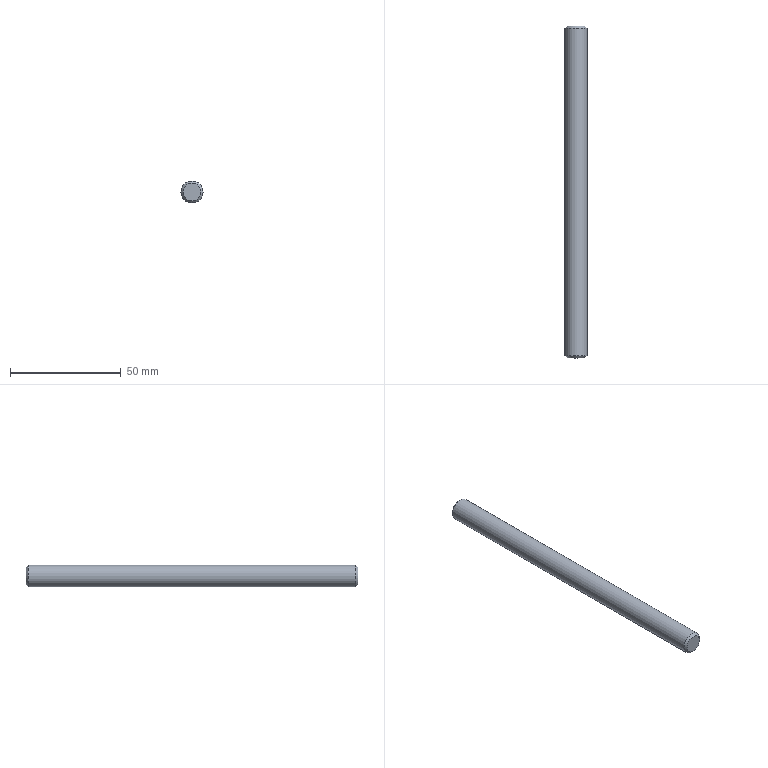Component | NX | REAMER_BAR | 1 solid | 5 faces | box 10 x 150 x 10 mm | volume 11752 mm3 | plane 2 | cone 2 | cylinder 1 | commonest cylinder face diameters 10 x1
STEP:
#1=CARTESIAN_POINT('',(0.,0.,0.));
#2=DIRECTION('',(0.,0.,1.));
#3=DIRECTION('',(1.,0.,0.));
#4=AXIS2_PLACEMENT_3D('',#1,#2,#3);
#5=CARTESIAN_POINT('',(-188.627,-125.996,15.));
#6=VERTEX_POINT('',#5);
#7=CARTESIAN_POINT('',(-192.627,-125.996,15.));
#8=DIRECTION('',(0.,-1.,0.));
#9=DIRECTION('',(1.,0.,0.));
#10=AXIS2_PLACEMENT_3D('',#7,#8,#9);
#11=CIRCLE('',#10,4.);
#12=CARTESIAN_POINT('',(-192.627,-125.996,15.));
#13=DIRECTION('',(0.,-1.,0.));
#14=DIRECTION('',(1.,0.,0.));
#15=AXIS2_PLACEMENT_3D('',#12,#13,#14);
#16=PLANE('',#15);
#17=CARTESIAN_POINT('',(0.,0.));
#18=DIRECTION('',(1.,0.));
#19=AXIS2_PLACEMENT_2D('',#17,#18);
#20=CIRCLE('',#19,4.);
#21=(GEOMETRIC_REPRESENTATION_CONTEXT(2)PARAMETRIC_REPRESENTATION_CONTEXT()REPRESENTATION_CONTEXT('',''));
#22=DEFINITIONAL_REPRESENTATION('',(#20),#21);
#23=PCURVE('',#16,#22);
#24=CARTESIAN_POINT('',(-192.627,-124.996,15.));
#25=DIRECTION('',(0.,1.,0.));
#26=DIRECTION('',(-1.,0.,0.));
#27=AXIS2_PLACEMENT_3D('',#24,#25,#26);
#28=CONICAL_SURFACE('',#27,5.,0.7854);
#29=CARTESIAN_POINT('',(9.425,-1.));
#30=DIRECTION('',(-1.,0.));
#31=VECTOR('',#30,1.);
#32=LINE('',#29,#31);
#33=(GEOMETRIC_REPRESENTATION_CONTEXT(2)PARAMETRIC_REPRESENTATION_CONTEXT()REPRESENTATION_CONTEXT('',''));
#34=DEFINITIONAL_REPRESENTATION('',(#32),#33);
#35=PCURVE('',#28,#34);
#36=SURFACE_CURVE('',#11,(#23,#35),.PCURVE_S1.);
#37=EDGE_CURVE('',#6,#6,#36,.T.);
#38=ORIENTED_EDGE('',*,*,#37,.T.);
#39=EDGE_LOOP('',(#38));
#40=FACE_BOUND('',#39,.T.);
#41=ADVANCED_FACE('',(#40),#16,.T.);
#42=CARTESIAN_POINT('',(-196.627,24.004,15.));
#43=VERTEX_POINT('',#42);
#44=CARTESIAN_POINT('',(-192.627,24.004,15.));
#45=DIRECTION('',(0.,1.,0.));
#46=DIRECTION('',(-1.,0.,0.));
#47=AXIS2_PLACEMENT_3D('',#44,#45,#46);
#48=CIRCLE('',#47,4.);
#49=CARTESIAN_POINT('',(-192.627,24.004,15.));
#50=DIRECTION('',(0.,1.,0.));
#51=DIRECTION('',(-1.,0.,0.));
#52=AXIS2_PLACEMENT_3D('',#49,#50,#51);
#53=PLANE('',#52);
#54=CARTESIAN_POINT('',(0.,0.));
#55=DIRECTION('',(1.,0.));
#56=AXIS2_PLACEMENT_2D('',#54,#55);
#57=CIRCLE('',#56,4.);
#58=(GEOMETRIC_REPRESENTATION_CONTEXT(2)PARAMETRIC_REPRESENTATION_CONTEXT()REPRESENTATION_CONTEXT('',''));
#59=DEFINITIONAL_REPRESENTATION('',(#57),#58);
#60=PCURVE('',#53,#59);
#61=CARTESIAN_POINT('',(-192.627,23.004,15.));
#62=DIRECTION('',(0.,-1.,0.));
#63=DIRECTION('',(1.,0.,0.));
#64=AXIS2_PLACEMENT_3D('',#61,#62,#63);
#65=CONICAL_SURFACE('',#64,5.,0.7854);
#66=CARTESIAN_POINT('',(9.425,-1.));
#67=DIRECTION('',(-1.,0.));
#68=VECTOR('',#67,1.);
#69=LINE('',#66,#68);
#70=(GEOMETRIC_REPRESENTATION_CONTEXT(2)PARAMETRIC_REPRESENTATION_CONTEXT()REPRESENTATION_CONTEXT('',''));
#71=DEFINITIONAL_REPRESENTATION('',(#69),#70);
#72=PCURVE('',#65,#71);
#73=SURFACE_CURVE('',#48,(#60,#72),.PCURVE_S1.);
#74=EDGE_CURVE('',#43,#43,#73,.T.);
#75=ORIENTED_EDGE('',*,*,#74,.T.);
#76=EDGE_LOOP('',(#75));
#77=FACE_BOUND('',#76,.T.);
#78=ADVANCED_FACE('',(#77),#53,.T.);
#79=CARTESIAN_POINT('',(-197.627,23.004,15.));
#80=VERTEX_POINT('',#79);
#81=CARTESIAN_POINT('',(-187.627,23.004,15.));
#82=VERTEX_POINT('',#81);
#83=CARTESIAN_POINT('',(-192.627,23.004,15.));
#84=DIRECTION('',(0.,-1.,0.));
#85=DIRECTION('',(-1.,0.,0.));
#86=AXIS2_PLACEMENT_3D('',#83,#84,#85);
#87=CIRCLE('',#86,5.);
#88=CARTESIAN_POINT('',(-192.627,24.004,15.));
#89=DIRECTION('',(0.,-1.,0.));
#90=DIRECTION('',(1.,0.,0.));
#91=AXIS2_PLACEMENT_3D('',#88,#89,#90);
#92=CYLINDRICAL_SURFACE('',#91,5.);
#93=CARTESIAN_POINT('',(3.142,1.));
#94=DIRECTION('',(1.,0.));
#95=VECTOR('',#94,1.);
#96=LINE('',#93,#95);
#97=(GEOMETRIC_REPRESENTATION_CONTEXT(2)PARAMETRIC_REPRESENTATION_CONTEXT()REPRESENTATION_CONTEXT('',''));
#98=DEFINITIONAL_REPRESENTATION('',(#96),#97);
#99=PCURVE('',#92,#98);
#100=CARTESIAN_POINT('',(3.142,0.));
#101=DIRECTION('',(1.,0.));
#102=VECTOR('',#101,1.);
#103=LINE('',#100,#102);
#104=(GEOMETRIC_REPRESENTATION_CONTEXT(2)PARAMETRIC_REPRESENTATION_CONTEXT()REPRESENTATION_CONTEXT('',''));
#105=DEFINITIONAL_REPRESENTATION('',(#103),#104);
#106=PCURVE('',#65,#105);
#107=SURFACE_CURVE('',#87,(#99,#106),.PCURVE_S1.);
#108=EDGE_CURVE('',#80,#82,#107,.T.);
#109=ORIENTED_EDGE('',*,*,#108,.T.);
#110=CARTESIAN_POINT('',(-187.627,-124.996,15.));
#111=VERTEX_POINT('',#110);
#112=CARTESIAN_POINT('',(-187.627,23.004,15.));
#113=CARTESIAN_POINT('',(-187.627,-124.996,15.));
#114=B_SPLINE_CURVE_WITH_KNOTS('',1,(#112,#113),.UNSPECIFIED.,.F.,.F.,(2,2),(1.,149.),.PIECEWISE_BEZIER_KNOTS.);
#115=CARTESIAN_POINT('',(6.283,0.));
#116=DIRECTION('',(0.,1.));
#117=VECTOR('',#116,1.);
#118=LINE('',#115,#117);
#119=(GEOMETRIC_REPRESENTATION_CONTEXT(2)PARAMETRIC_REPRESENTATION_CONTEXT()REPRESENTATION_CONTEXT('',''));
#120=DEFINITIONAL_REPRESENTATION('',(#118),#119);
#121=PCURVE('',#92,#120);
#122=CARTESIAN_POINT('',(0.,0.));
#123=DIRECTION('',(0.,1.));
#124=VECTOR('',#123,1.);
#125=LINE('',#122,#124);
#126=(GEOMETRIC_REPRESENTATION_CONTEXT(2)PARAMETRIC_REPRESENTATION_CONTEXT()REPRESENTATION_CONTEXT('',''));
#127=DEFINITIONAL_REPRESENTATION('',(#125),#126);
#128=PCURVE('',#92,#127);
#129=SEAM_CURVE('',#114,(#121,#128),.PCURVE_S1.);
#130=EDGE_CURVE('',#82,#111,#129,.T.);
#131=ORIENTED_EDGE('',*,*,#130,.T.);
#132=CARTESIAN_POINT('',(-192.627,-124.996,15.));
#133=DIRECTION('',(0.,1.,0.));
#134=DIRECTION('',(1.,0.,0.));
#135=AXIS2_PLACEMENT_3D('',#132,#133,#134);
#136=CIRCLE('',#135,5.);
#137=CARTESIAN_POINT('',(6.283,149.));
#138=DIRECTION('',(-1.,0.));
#139=VECTOR('',#138,1.);
#140=LINE('',#137,#139);
#141=(GEOMETRIC_REPRESENTATION_CONTEXT(2)PARAMETRIC_REPRESENTATION_CONTEXT()REPRESENTATION_CONTEXT('',''));
#142=DEFINITIONAL_REPRESENTATION('',(#140),#141);
#143=PCURVE('',#92,#142);
#144=CARTESIAN_POINT('',(3.142,0.));
#145=DIRECTION('',(1.,0.));
#146=VECTOR('',#145,1.);
#147=LINE('',#144,#146);
#148=(GEOMETRIC_REPRESENTATION_CONTEXT(2)PARAMETRIC_REPRESENTATION_CONTEXT()REPRESENTATION_CONTEXT('',''));
#149=DEFINITIONAL_REPRESENTATION('',(#147),#148);
#150=PCURVE('',#28,#149);
#151=SURFACE_CURVE('',#136,(#143,#150),.PCURVE_S1.);
#152=EDGE_CURVE('',#111,#111,#151,.T.);
#153=ORIENTED_EDGE('',*,*,#152,.T.);
#154=ORIENTED_EDGE('',*,*,#130,.F.);
#155=CARTESIAN_POINT('',(-192.627,23.004,15.));
#156=DIRECTION('',(0.,-1.,0.));
#157=DIRECTION('',(-1.,0.,0.));
#158=AXIS2_PLACEMENT_3D('',#155,#156,#157);
#159=CIRCLE('',#158,5.);
#160=CARTESIAN_POINT('',(-3.142,1.));
#161=DIRECTION('',(1.,0.));
#162=VECTOR('',#161,1.);
#163=LINE('',#160,#162);
#164=(GEOMETRIC_REPRESENTATION_CONTEXT(2)PARAMETRIC_REPRESENTATION_CONTEXT()REPRESENTATION_CONTEXT('',''));
#165=DEFINITIONAL_REPRESENTATION('',(#163),#164);
#166=PCURVE('',#92,#165);
#167=CARTESIAN_POINT('',(3.142,0.));
#168=DIRECTION('',(1.,0.));
#169=VECTOR('',#168,1.);
#170=LINE('',#167,#169);
#171=(GEOMETRIC_REPRESENTATION_CONTEXT(2)PARAMETRIC_REPRESENTATION_CONTEXT()REPRESENTATION_CONTEXT('',''));
#172=DEFINITIONAL_REPRESENTATION('',(#170),#171);
#173=PCURVE('',#65,#172);
#174=SURFACE_CURVE('',#159,(#166,#173),.PCURVE_S1.);
#175=EDGE_CURVE('',#82,#80,#174,.T.);
#176=ORIENTED_EDGE('',*,*,#175,.T.);
#177=EDGE_LOOP('',(#109,#131,#153,#154,#176));
#178=FACE_BOUND('',#177,.T.);
#179=ADVANCED_FACE('',(#178),#92,.T.);
#180=ORIENTED_EDGE('',*,*,#74,.F.);
#181=CARTESIAN_POINT('',(-196.627,24.004,15.));
#182=CARTESIAN_POINT('',(-197.627,23.004,15.));
#183=B_SPLINE_CURVE_WITH_KNOTS('',1,(#181,#182),.UNSPECIFIED.,.F.,.F.,(2,2),(-1.414,0.),.PIECEWISE_BEZIER_KNOTS.);
#184=CARTESIAN_POINT('',(9.425,0.));
#185=DIRECTION('',(0.,1.));
#186=VECTOR('',#185,1.);
#187=LINE('',#184,#186);
#188=(GEOMETRIC_REPRESENTATION_CONTEXT(2)PARAMETRIC_REPRESENTATION_CONTEXT()REPRESENTATION_CONTEXT('',''));
#189=DEFINITIONAL_REPRESENTATION('',(#187),#188);
#190=PCURVE('',#65,#189);
#191=CARTESIAN_POINT('',(3.142,0.));
#192=DIRECTION('',(0.,1.));
#193=VECTOR('',#192,1.);
#194=LINE('',#191,#193);
#195=(GEOMETRIC_REPRESENTATION_CONTEXT(2)PARAMETRIC_REPRESENTATION_CONTEXT()REPRESENTATION_CONTEXT('',''));
#196=DEFINITIONAL_REPRESENTATION('',(#194),#195);
#197=PCURVE('',#65,#196);
#198=SEAM_CURVE('',#183,(#190,#197),.PCURVE_S1.);
#199=EDGE_CURVE('',#43,#80,#198,.T.);
#200=ORIENTED_EDGE('',*,*,#199,.T.);
#201=ORIENTED_EDGE('',*,*,#175,.F.);
#202=ORIENTED_EDGE('',*,*,#108,.F.);
#203=ORIENTED_EDGE('',*,*,#199,.F.);
#204=EDGE_LOOP('',(#180,#200,#201,#202,#203));
#205=FACE_BOUND('',#204,.T.);
#206=ADVANCED_FACE('',(#205),#65,.T.);
#207=ORIENTED_EDGE('',*,*,#37,.F.);
#208=CARTESIAN_POINT('',(-188.627,-125.996,15.));
#209=CARTESIAN_POINT('',(-187.627,-124.996,15.));
#210=B_SPLINE_CURVE_WITH_KNOTS('',1,(#208,#209),.UNSPECIFIED.,.F.,.F.,(2,2),(-1.414,0.),.PIECEWISE_BEZIER_KNOTS.);
#211=CARTESIAN_POINT('',(9.425,0.));
#212=DIRECTION('',(0.,1.));
#213=VECTOR('',#212,1.);
#214=LINE('',#211,#213);
#215=(GEOMETRIC_REPRESENTATION_CONTEXT(2)PARAMETRIC_REPRESENTATION_CONTEXT()REPRESENTATION_CONTEXT('',''));
#216=DEFINITIONAL_REPRESENTATION('',(#214),#215);
#217=PCURVE('',#28,#216);
#218=CARTESIAN_POINT('',(3.142,0.));
#219=DIRECTION('',(0.,1.));
#220=VECTOR('',#219,1.);
#221=LINE('',#218,#220);
#222=(GEOMETRIC_REPRESENTATION_CONTEXT(2)PARAMETRIC_REPRESENTATION_CONTEXT()REPRESENTATION_CONTEXT('',''));
#223=DEFINITIONAL_REPRESENTATION('',(#221),#222);
#224=PCURVE('',#28,#223);
#225=SEAM_CURVE('',#210,(#217,#224),.PCURVE_S1.);
#226=EDGE_CURVE('',#6,#111,#225,.T.);
#227=ORIENTED_EDGE('',*,*,#226,.T.);
#228=ORIENTED_EDGE('',*,*,#152,.F.);
#229=ORIENTED_EDGE('',*,*,#226,.F.);
#230=EDGE_LOOP('',(#207,#227,#228,#229));
#231=FACE_BOUND('',#230,.T.);
#232=ADVANCED_FACE('',(#231),#28,.T.);
#233=CLOSED_SHELL('',(#41,#78,#179,#206,#232));
#234=MANIFOLD_SOLID_BREP('',#233);
#235=(LENGTH_UNIT()NAMED_UNIT(*)SI_UNIT(.MILLI.,.METRE.));
#236=UNCERTAINTY_MEASURE_WITH_UNIT(LENGTH_MEASURE(0.00001),#235,'','');
#237=(NAMED_UNIT(*)PLANE_ANGLE_UNIT()SI_UNIT($,.RADIAN.));
#238=(NAMED_UNIT(*)SI_UNIT($,.STERADIAN.)SOLID_ANGLE_UNIT());
#239=(GEOMETRIC_REPRESENTATION_CONTEXT(3)GLOBAL_UNCERTAINTY_ASSIGNED_CONTEXT((#236))GLOBAL_UNIT_ASSIGNED_CONTEXT((#235,#237,#238))REPRESENTATION_CONTEXT('',''));
#240=ADVANCED_BREP_SHAPE_REPRESENTATION('',(#4,#234),#239);